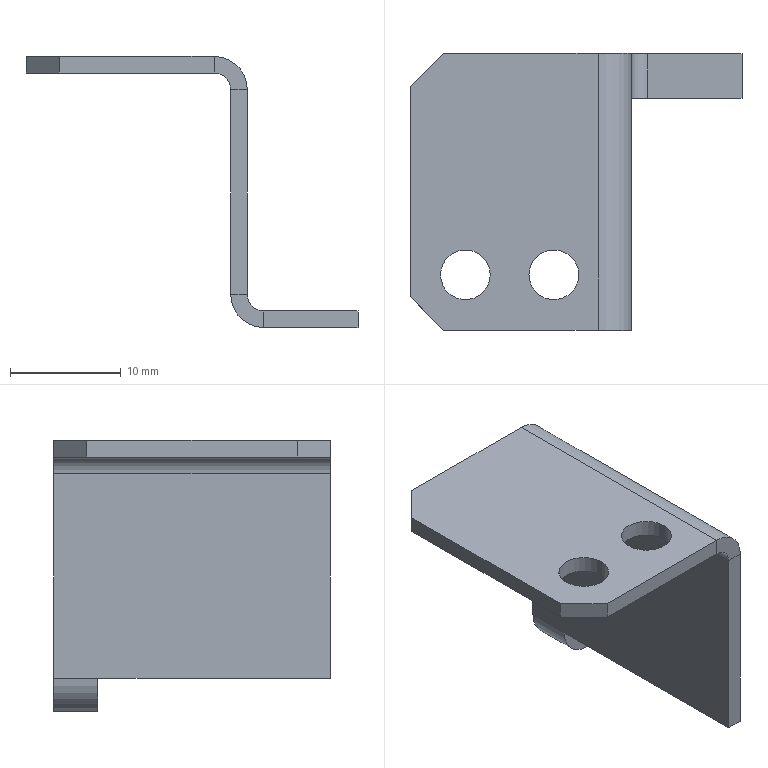Component | SolidWorks | F12529-S5109-1 | 1 solid | 29 faces | box 30 x 25 x 24.5 mm | volume 1475 mm3 | plane 21 | cylinder 8 | commonest cylinder face diameters 4.5 x4 6 x2 3 x2
STEP:
#1=CARTESIAN_POINT('',(-1.467,7.795,-1.201));
#2=VERTEX_POINT('',#1);
#3=CARTESIAN_POINT('',(-1.644,7.795,-1.201));
#4=VERTEX_POINT('',#3);
#5=CARTESIAN_POINT('',(-1.555,7.795,-1.201));
#6=DIRECTION('',(-0.,-0.,1.));
#7=DIRECTION('',(-1.,0.,-0.));
#8=AXIS2_PLACEMENT_3D('',#5,#6,#7);
#9=CIRCLE('',#8,0.08858);
#10=EDGE_CURVE('',#2,#4,#9,.T.);
#11=ORIENTED_EDGE('',*,*,#10,.T.);
#12=CARTESIAN_POINT('',(-1.644,7.795,-1.26));
#13=VERTEX_POINT('',#12);
#14=CARTESIAN_POINT('',(-1.644,7.795,-0.8661));
#15=DIRECTION('',(0.,0.,-1.));
#16=VECTOR('',#15,39.37);
#17=LINE('',#14,#16);
#18=EDGE_CURVE('',#4,#13,#17,.T.);
#19=ORIENTED_EDGE('',*,*,#18,.T.);
#20=CARTESIAN_POINT('',(-1.467,7.795,-1.26));
#21=VERTEX_POINT('',#20);
#22=CARTESIAN_POINT('',(-1.555,7.795,-1.26));
#23=DIRECTION('',(0.,0.,-1.));
#24=DIRECTION('',(1.,0.,0.));
#25=AXIS2_PLACEMENT_3D('',#22,#23,#24);
#26=CIRCLE('',#25,0.08858);
#27=EDGE_CURVE('',#13,#21,#26,.T.);
#28=ORIENTED_EDGE('',*,*,#27,.T.);
#29=CARTESIAN_POINT('',(-1.467,7.795,-0.8661));
#30=DIRECTION('',(0.,0.,-1.));
#31=VECTOR('',#30,39.37);
#32=LINE('',#29,#31);
#33=EDGE_CURVE('',#2,#21,#32,.T.);
#34=ORIENTED_EDGE('',*,*,#33,.F.);
#35=EDGE_LOOP('',(#11,#19,#28,#34));
#36=FACE_OUTER_BOUND('',#35,.T.);
#37=CARTESIAN_POINT('',(-1.555,7.795,-0.8661));
#38=DIRECTION('',(0.,0.,-1.));
#39=DIRECTION('',(1.,0.,0.));
#40=AXIS2_PLACEMENT_3D('',#37,#38,#39);
#41=CYLINDRICAL_SURFACE('',#40,0.08858);
#42=ADVANCED_FACE('',(#36),#41,.F.);
#43=CARTESIAN_POINT('',(-1.781,7.795,-1.201));
#44=VERTEX_POINT('',#43);
#45=CARTESIAN_POINT('',(-1.959,7.795,-1.201));
#46=VERTEX_POINT('',#45);
#47=CARTESIAN_POINT('',(-1.87,7.795,-1.201));
#48=DIRECTION('',(-0.,-0.,1.));
#49=DIRECTION('',(-1.,0.,-0.));
#50=AXIS2_PLACEMENT_3D('',#47,#48,#49);
#51=CIRCLE('',#50,0.08858);
#52=EDGE_CURVE('',#44,#46,#51,.T.);
#53=ORIENTED_EDGE('',*,*,#52,.T.);
#54=CARTESIAN_POINT('',(-1.959,7.795,-1.26));
#55=VERTEX_POINT('',#54);
#56=CARTESIAN_POINT('',(-1.959,7.795,-0.8661));
#57=DIRECTION('',(0.,0.,-1.));
#58=VECTOR('',#57,39.37);
#59=LINE('',#56,#58);
#60=EDGE_CURVE('',#46,#55,#59,.T.);
#61=ORIENTED_EDGE('',*,*,#60,.T.);
#62=CARTESIAN_POINT('',(-1.781,7.795,-1.26));
#63=VERTEX_POINT('',#62);
#64=CARTESIAN_POINT('',(-1.87,7.795,-1.26));
#65=DIRECTION('',(0.,0.,-1.));
#66=DIRECTION('',(1.,0.,0.));
#67=AXIS2_PLACEMENT_3D('',#64,#65,#66);
#68=CIRCLE('',#67,0.08858);
#69=EDGE_CURVE('',#55,#63,#68,.T.);
#70=ORIENTED_EDGE('',*,*,#69,.T.);
#71=CARTESIAN_POINT('',(-1.781,7.795,-0.8661));
#72=DIRECTION('',(0.,0.,-1.));
#73=VECTOR('',#72,39.37);
#74=LINE('',#71,#73);
#75=EDGE_CURVE('',#44,#63,#74,.T.);
#76=ORIENTED_EDGE('',*,*,#75,.F.);
#77=EDGE_LOOP('',(#53,#61,#70,#76));
#78=FACE_OUTER_BOUND('',#77,.T.);
#79=CARTESIAN_POINT('',(-1.87,7.795,-0.8661));
#80=DIRECTION('',(0.,0.,-1.));
#81=DIRECTION('',(1.,0.,0.));
#82=AXIS2_PLACEMENT_3D('',#79,#80,#81);
#83=CYLINDRICAL_SURFACE('',#82,0.08858);
#84=ADVANCED_FACE('',(#78),#83,.F.);
#85=CARTESIAN_POINT('',(-1.28,7.598,-1.319));
#86=VERTEX_POINT('',#85);
#87=CARTESIAN_POINT('',(-1.339,7.598,-1.319));
#88=VERTEX_POINT('',#87);
#89=CARTESIAN_POINT('',(-1.28,7.598,-1.319));
#90=DIRECTION('',(-1.,-0.,-0.));
#91=VECTOR('',#90,39.37);
#92=LINE('',#89,#91);
#93=EDGE_CURVE('',#86,#88,#92,.T.);
#94=ORIENTED_EDGE('',*,*,#93,.F.);
#95=CARTESIAN_POINT('',(-1.398,7.598,-1.201));
#96=VERTEX_POINT('',#95);
#97=CARTESIAN_POINT('',(-1.398,7.598,-1.319));
#98=DIRECTION('',(-0.,1.,-0.));
#99=DIRECTION('',(-1.,0.,0.));
#100=AXIS2_PLACEMENT_3D('',#97,#98,#99);
#101=CIRCLE('',#100,0.1181);
#102=EDGE_CURVE('',#96,#86,#101,.T.);
#103=ORIENTED_EDGE('',*,*,#102,.F.);
#104=CARTESIAN_POINT('',(-1.398,7.598,-1.26));
#105=VERTEX_POINT('',#104);
#106=CARTESIAN_POINT('',(-1.398,7.598,-1.26));
#107=DIRECTION('',(-0.,-0.,1.));
#108=VECTOR('',#107,39.37);
#109=LINE('',#106,#108);
#110=EDGE_CURVE('',#105,#96,#109,.T.);
#111=ORIENTED_EDGE('',*,*,#110,.F.);
#112=CARTESIAN_POINT('',(-1.398,7.598,-1.319));
#113=DIRECTION('',(-0.,1.,-0.));
#114=DIRECTION('',(0.,0.,-1.));
#115=AXIS2_PLACEMENT_3D('',#112,#113,#114);
#116=CIRCLE('',#115,0.05906);
#117=EDGE_CURVE('',#105,#88,#116,.T.);
#118=ORIENTED_EDGE('',*,*,#117,.T.);
#119=EDGE_LOOP('',(#94,#103,#111,#118));
#120=FACE_OUTER_BOUND('',#119,.T.);
#121=CARTESIAN_POINT('',(-1.28,7.598,-1.319));
#122=DIRECTION('',(0.,-1.,0.));
#123=DIRECTION('',(-1.,-0.,-0.));
#124=AXIS2_PLACEMENT_3D('',#121,#122,#123);
#125=PLANE('',#124);
#126=ADVANCED_FACE('',(#120),#125,.T.);
#127=CARTESIAN_POINT('',(-1.28,7.598,-2.047));
#128=VERTEX_POINT('',#127);
#129=CARTESIAN_POINT('',(-1.28,7.598,-1.201));
#130=DIRECTION('',(0.,0.,-1.));
#131=VECTOR('',#130,39.37);
#132=LINE('',#129,#131);
#133=EDGE_CURVE('',#86,#128,#132,.T.);
#134=ORIENTED_EDGE('',*,*,#133,.F.);
#135=ORIENTED_EDGE('',*,*,#93,.T.);
#136=CARTESIAN_POINT('',(-1.339,7.598,-2.047));
#137=VERTEX_POINT('',#136);
#138=CARTESIAN_POINT('',(-1.339,7.598,-1.201));
#139=DIRECTION('',(0.,0.,-1.));
#140=VECTOR('',#139,39.37);
#141=LINE('',#138,#140);
#142=EDGE_CURVE('',#88,#137,#141,.T.);
#143=ORIENTED_EDGE('',*,*,#142,.T.);
#144=CARTESIAN_POINT('',(-1.339,7.598,-2.047));
#145=DIRECTION('',(1.,0.,0.));
#146=VECTOR('',#145,39.37);
#147=LINE('',#144,#146);
#148=EDGE_CURVE('',#137,#128,#147,.T.);
#149=ORIENTED_EDGE('',*,*,#148,.T.);
#150=EDGE_LOOP('',(#134,#135,#143,#149));
#151=FACE_OUTER_BOUND('',#150,.T.);
#152=CARTESIAN_POINT('',(-1.398,7.598,-1.26));
#153=DIRECTION('',(0.,-1.,0.));
#154=DIRECTION('',(-1.,-0.,-0.));
#155=AXIS2_PLACEMENT_3D('',#152,#153,#154);
#156=PLANE('',#155);
#157=ADVANCED_FACE('',(#151),#156,.T.);
#158=CARTESIAN_POINT('',(-1.398,8.583,-1.201));
#159=VERTEX_POINT('',#158);
#160=CARTESIAN_POINT('',(-1.398,8.583,-1.26));
#161=VERTEX_POINT('',#160);
#162=CARTESIAN_POINT('',(-1.398,8.583,-1.201));
#163=DIRECTION('',(0.,0.,-1.));
#164=VECTOR('',#163,39.37);
#165=LINE('',#162,#164);
#166=EDGE_CURVE('',#159,#161,#165,.T.);
#167=ORIENTED_EDGE('',*,*,#166,.F.);
#168=CARTESIAN_POINT('',(-1.28,8.583,-1.319));
#169=VERTEX_POINT('',#168);
#170=CARTESIAN_POINT('',(-1.398,8.583,-1.319));
#171=DIRECTION('',(-0.,1.,-0.));
#172=DIRECTION('',(-1.,0.,-0.));
#173=AXIS2_PLACEMENT_3D('',#170,#171,#172);
#174=CIRCLE('',#173,0.1181);
#175=EDGE_CURVE('',#159,#169,#174,.T.);
#176=ORIENTED_EDGE('',*,*,#175,.T.);
#177=CARTESIAN_POINT('',(-1.339,8.583,-1.319));
#178=VERTEX_POINT('',#177);
#179=CARTESIAN_POINT('',(-1.339,8.583,-1.319));
#180=DIRECTION('',(1.,0.,0.));
#181=VECTOR('',#180,39.37);
#182=LINE('',#179,#181);
#183=EDGE_CURVE('',#178,#169,#182,.T.);
#184=ORIENTED_EDGE('',*,*,#183,.F.);
#185=CARTESIAN_POINT('',(-1.398,8.583,-1.319));
#186=DIRECTION('',(-0.,1.,-0.));
#187=DIRECTION('',(0.,0.,-1.));
#188=AXIS2_PLACEMENT_3D('',#185,#186,#187);
#189=CIRCLE('',#188,0.05906);
#190=EDGE_CURVE('',#161,#178,#189,.T.);
#191=ORIENTED_EDGE('',*,*,#190,.F.);
#192=EDGE_LOOP('',(#167,#176,#184,#191));
#193=FACE_OUTER_BOUND('',#192,.T.);
#194=CARTESIAN_POINT('',(-1.398,8.583,-1.201));
#195=DIRECTION('',(-0.,1.,-0.));
#196=DIRECTION('',(1.,0.,0.));
#197=AXIS2_PLACEMENT_3D('',#194,#195,#196);
#198=PLANE('',#197);
#199=ADVANCED_FACE('',(#193),#198,.T.);
#200=CARTESIAN_POINT('',(-1.949,8.583,-1.26));
#201=VERTEX_POINT('',#200);
#202=CARTESIAN_POINT('',(-2.067,8.583,-1.26));
#203=DIRECTION('',(1.,0.,0.));
#204=VECTOR('',#203,39.37);
#205=LINE('',#202,#204);
#206=EDGE_CURVE('',#201,#161,#205,.T.);
#207=ORIENTED_EDGE('',*,*,#206,.F.);
#208=CARTESIAN_POINT('',(-1.949,8.583,-1.201));
#209=VERTEX_POINT('',#208);
#210=CARTESIAN_POINT('',(-1.949,8.583,-1.319));
#211=DIRECTION('',(-0.,-0.,1.));
#212=VECTOR('',#211,39.37);
#213=LINE('',#210,#212);
#214=EDGE_CURVE('',#201,#209,#213,.T.);
#215=ORIENTED_EDGE('',*,*,#214,.T.);
#216=CARTESIAN_POINT('',(-2.067,8.583,-1.201));
#217=DIRECTION('',(1.,0.,0.));
#218=VECTOR('',#217,39.37);
#219=LINE('',#216,#218);
#220=EDGE_CURVE('',#209,#159,#219,.T.);
#221=ORIENTED_EDGE('',*,*,#220,.T.);
#222=ORIENTED_EDGE('',*,*,#166,.T.);
#223=EDGE_LOOP('',(#207,#215,#221,#222));
#224=FACE_OUTER_BOUND('',#223,.T.);
#225=CARTESIAN_POINT('',(-1.339,8.583,-1.319));
#226=DIRECTION('',(-0.,1.,-0.));
#227=DIRECTION('',(1.,0.,0.));
#228=AXIS2_PLACEMENT_3D('',#225,#226,#227);
#229=PLANE('',#228);
#230=ADVANCED_FACE('',(#224),#229,.T.);
#231=CARTESIAN_POINT('',(-1.28,8.583,-2.047));
#232=VERTEX_POINT('',#231);
#233=CARTESIAN_POINT('',(-1.28,8.583,-1.201));
#234=DIRECTION('',(0.,0.,-1.));
#235=VECTOR('',#234,39.37);
#236=LINE('',#233,#235);
#237=EDGE_CURVE('',#169,#232,#236,.T.);
#238=ORIENTED_EDGE('',*,*,#237,.T.);
#239=CARTESIAN_POINT('',(-1.339,8.583,-2.047));
#240=VERTEX_POINT('',#239);
#241=CARTESIAN_POINT('',(-1.28,8.583,-2.047));
#242=DIRECTION('',(-1.,-0.,-0.));
#243=VECTOR('',#242,39.37);
#244=LINE('',#241,#243);
#245=EDGE_CURVE('',#232,#240,#244,.T.);
#246=ORIENTED_EDGE('',*,*,#245,.T.);
#247=CARTESIAN_POINT('',(-1.339,8.583,-1.201));
#248=DIRECTION('',(0.,0.,-1.));
#249=VECTOR('',#248,39.37);
#250=LINE('',#247,#249);
#251=EDGE_CURVE('',#178,#240,#250,.T.);
#252=ORIENTED_EDGE('',*,*,#251,.F.);
#253=ORIENTED_EDGE('',*,*,#183,.T.);
#254=EDGE_LOOP('',(#238,#246,#252,#253));
#255=FACE_OUTER_BOUND('',#254,.T.);
#256=CARTESIAN_POINT('',(-1.22,8.583,-2.165));
#257=DIRECTION('',(-0.,1.,-0.));
#258=DIRECTION('',(1.,0.,0.));
#259=AXIS2_PLACEMENT_3D('',#256,#257,#258);
#260=PLANE('',#259);
#261=ADVANCED_FACE('',(#255),#260,.T.);
#262=ORIENTED_EDGE('',*,*,#237,.F.);
#263=CARTESIAN_POINT('',(-1.28,7.598,-1.319));
#264=DIRECTION('',(-0.,1.,-0.));
#265=VECTOR('',#264,39.37);
#266=LINE('',#263,#265);
#267=EDGE_CURVE('',#86,#169,#266,.T.);
#268=ORIENTED_EDGE('',*,*,#267,.F.);
#269=ORIENTED_EDGE('',*,*,#133,.T.);
#270=CARTESIAN_POINT('',(-1.28,8.425,-2.047));
#271=VERTEX_POINT('',#270);
#272=CARTESIAN_POINT('',(-1.28,7.598,-2.047));
#273=DIRECTION('',(-0.,1.,-0.));
#274=VECTOR('',#273,39.37);
#275=LINE('',#272,#274);
#276=EDGE_CURVE('',#128,#271,#275,.T.);
#277=ORIENTED_EDGE('',*,*,#276,.T.);
#278=CARTESIAN_POINT('',(-1.28,7.598,-2.047));
#279=DIRECTION('',(-0.,1.,-0.));
#280=VECTOR('',#279,39.37);
#281=LINE('',#278,#280);
#282=EDGE_CURVE('',#271,#232,#281,.T.);
#283=ORIENTED_EDGE('',*,*,#282,.T.);
#284=EDGE_LOOP('',(#262,#268,#269,#277,#283));
#285=FACE_OUTER_BOUND('',#284,.T.);
#286=CARTESIAN_POINT('',(-1.28,7.598,-1.201));
#287=DIRECTION('',(1.,0.,0.));
#288=DIRECTION('',(-0.,-0.,1.));
#289=AXIS2_PLACEMENT_3D('',#286,#287,#288);
#290=PLANE('',#289);
#291=ADVANCED_FACE('',(#285),#290,.T.);
#292=ORIENTED_EDGE('',*,*,#175,.F.);
#293=CARTESIAN_POINT('',(-1.398,7.598,-1.201));
#294=DIRECTION('',(-0.,1.,-0.));
#295=VECTOR('',#294,39.37);
#296=LINE('',#293,#295);
#297=EDGE_CURVE('',#96,#159,#296,.T.);
#298=ORIENTED_EDGE('',*,*,#297,.F.);
#299=ORIENTED_EDGE('',*,*,#102,.T.);
#300=ORIENTED_EDGE('',*,*,#267,.T.);
#301=EDGE_LOOP('',(#292,#298,#299,#300));
#302=FACE_OUTER_BOUND('',#301,.T.);
#303=CARTESIAN_POINT('',(-1.398,7.598,-1.319));
#304=DIRECTION('',(-0.,1.,-0.));
#305=DIRECTION('',(1.,0.,0.));
#306=AXIS2_PLACEMENT_3D('',#303,#304,#305);
#307=CYLINDRICAL_SURFACE('',#306,0.1181);
#308=ADVANCED_FACE('',(#302),#307,.T.);
#309=ORIENTED_EDGE('',*,*,#10,.F.);
#310=CARTESIAN_POINT('',(-1.555,7.795,-1.201));
#311=DIRECTION('',(-0.,-0.,1.));
#312=DIRECTION('',(-1.,0.,-0.));
#313=AXIS2_PLACEMENT_3D('',#310,#311,#312);
#314=CIRCLE('',#313,0.08858);
#315=EDGE_CURVE('',#4,#2,#314,.T.);
#316=ORIENTED_EDGE('',*,*,#315,.F.);
#317=EDGE_LOOP('',(#309,#316));
#318=FACE_BOUND('',#317,.T.);
#319=ORIENTED_EDGE('',*,*,#52,.F.);
#320=CARTESIAN_POINT('',(-1.87,7.795,-1.201));
#321=DIRECTION('',(-0.,-0.,1.));
#322=DIRECTION('',(-1.,0.,-0.));
#323=AXIS2_PLACEMENT_3D('',#320,#321,#322);
#324=CIRCLE('',#323,0.08858);
#325=EDGE_CURVE('',#46,#44,#324,.T.);
#326=ORIENTED_EDGE('',*,*,#325,.F.);
#327=EDGE_LOOP('',(#319,#326));
#328=FACE_BOUND('',#327,.T.);
#329=ORIENTED_EDGE('',*,*,#220,.F.);
#330=CARTESIAN_POINT('',(-2.067,8.465,-1.201));
#331=VERTEX_POINT('',#330);
#332=CARTESIAN_POINT('',(-2.5,8.031,-1.201));
#333=DIRECTION('',(-0.7071,-0.7071,-0.));
#334=VECTOR('',#333,39.37);
#335=LINE('',#332,#334);
#336=EDGE_CURVE('',#209,#331,#335,.T.);
#337=ORIENTED_EDGE('',*,*,#336,.T.);
#338=CARTESIAN_POINT('',(-2.067,7.717,-1.201));
#339=VERTEX_POINT('',#338);
#340=CARTESIAN_POINT('',(-2.067,7.598,-1.201));
#341=DIRECTION('',(-0.,1.,-0.));
#342=VECTOR('',#341,39.37);
#343=LINE('',#340,#342);
#344=EDGE_CURVE('',#339,#331,#343,.T.);
#345=ORIENTED_EDGE('',*,*,#344,.F.);
#346=CARTESIAN_POINT('',(-1.949,7.598,-1.201));
#347=VERTEX_POINT('',#346);
#348=CARTESIAN_POINT('',(-2.008,7.657,-1.201));
#349=DIRECTION('',(0.7071,-0.7071,0.));
#350=VECTOR('',#349,39.37);
#351=LINE('',#348,#350);
#352=EDGE_CURVE('',#339,#347,#351,.T.);
#353=ORIENTED_EDGE('',*,*,#352,.T.);
#354=CARTESIAN_POINT('',(-2.067,7.598,-1.201));
#355=DIRECTION('',(1.,0.,0.));
#356=VECTOR('',#355,39.37);
#357=LINE('',#354,#356);
#358=EDGE_CURVE('',#347,#96,#357,.T.);
#359=ORIENTED_EDGE('',*,*,#358,.T.);
#360=ORIENTED_EDGE('',*,*,#297,.T.);
#361=EDGE_LOOP('',(#329,#337,#345,#353,#359,#360));
#362=FACE_OUTER_BOUND('',#361,.T.);
#363=CARTESIAN_POINT('',(-2.067,7.598,-1.201));
#364=DIRECTION('',(-0.,-0.,1.));
#365=DIRECTION('',(-1.,-0.,-0.));
#366=AXIS2_PLACEMENT_3D('',#363,#364,#365);
#367=PLANE('',#366);
#368=ADVANCED_FACE('',(#318,#328,#362),#367,.T.);
#369=ORIENTED_EDGE('',*,*,#344,.T.);
#370=CARTESIAN_POINT('',(-2.067,8.465,-1.26));
#371=VERTEX_POINT('',#370);
#372=CARTESIAN_POINT('',(-2.067,8.465,-1.26));
#373=DIRECTION('',(0.,0.,-1.));
#374=VECTOR('',#373,39.37);
#375=LINE('',#372,#374);
#376=EDGE_CURVE('',#331,#371,#375,.T.);
#377=ORIENTED_EDGE('',*,*,#376,.T.);
#378=CARTESIAN_POINT('',(-2.067,7.717,-1.26));
#379=VERTEX_POINT('',#378);
#380=CARTESIAN_POINT('',(-2.067,7.598,-1.26));
#381=DIRECTION('',(-0.,1.,-0.));
#382=VECTOR('',#381,39.37);
#383=LINE('',#380,#382);
#384=EDGE_CURVE('',#379,#371,#383,.T.);
#385=ORIENTED_EDGE('',*,*,#384,.F.);
#386=CARTESIAN_POINT('',(-2.067,7.717,-1.201));
#387=DIRECTION('',(-0.,-0.,1.));
#388=VECTOR('',#387,39.37);
#389=LINE('',#386,#388);
#390=EDGE_CURVE('',#379,#339,#389,.T.);
#391=ORIENTED_EDGE('',*,*,#390,.T.);
#392=EDGE_LOOP('',(#369,#377,#385,#391));
#393=FACE_OUTER_BOUND('',#392,.T.);
#394=CARTESIAN_POINT('',(-2.067,7.598,-1.26));
#395=DIRECTION('',(-1.,-0.,-0.));
#396=DIRECTION('',(0.,0.,-1.));
#397=AXIS2_PLACEMENT_3D('',#394,#395,#396);
#398=PLANE('',#397);
#399=ADVANCED_FACE('',(#393),#398,.T.);
#400=CARTESIAN_POINT('',(-1.555,7.795,-1.26));
#401=DIRECTION('',(0.,0.,-1.));
#402=DIRECTION('',(1.,0.,0.));
#403=AXIS2_PLACEMENT_3D('',#400,#401,#402);
#404=CIRCLE('',#403,0.08858);
#405=EDGE_CURVE('',#21,#13,#404,.T.);
#406=ORIENTED_EDGE('',*,*,#405,.F.);
#407=ORIENTED_EDGE('',*,*,#27,.F.);
#408=EDGE_LOOP('',(#406,#407));
#409=FACE_BOUND('',#408,.T.);
#410=CARTESIAN_POINT('',(-1.87,7.795,-1.26));
#411=DIRECTION('',(0.,0.,-1.));
#412=DIRECTION('',(1.,0.,0.));
#413=AXIS2_PLACEMENT_3D('',#410,#411,#412);
#414=CIRCLE('',#413,0.08858);
#415=EDGE_CURVE('',#63,#55,#414,.T.);
#416=ORIENTED_EDGE('',*,*,#415,.F.);
#417=ORIENTED_EDGE('',*,*,#69,.F.);
#418=EDGE_LOOP('',(#416,#417));
#419=FACE_BOUND('',#418,.T.);
#420=ORIENTED_EDGE('',*,*,#384,.T.);
#421=CARTESIAN_POINT('',(-1.949,8.583,-1.26));
#422=DIRECTION('',(0.7071,0.7071,0.));
#423=VECTOR('',#422,39.37);
#424=LINE('',#421,#423);
#425=EDGE_CURVE('',#371,#201,#424,.T.);
#426=ORIENTED_EDGE('',*,*,#425,.T.);
#427=ORIENTED_EDGE('',*,*,#206,.T.);
#428=CARTESIAN_POINT('',(-1.398,7.598,-1.26));
#429=DIRECTION('',(-0.,1.,-0.));
#430=VECTOR('',#429,39.37);
#431=LINE('',#428,#430);
#432=EDGE_CURVE('',#105,#161,#431,.T.);
#433=ORIENTED_EDGE('',*,*,#432,.F.);
#434=CARTESIAN_POINT('',(-1.949,7.598,-1.26));
#435=VERTEX_POINT('',#434);
#436=CARTESIAN_POINT('',(-2.067,7.598,-1.26));
#437=DIRECTION('',(1.,0.,0.));
#438=VECTOR('',#437,39.37);
#439=LINE('',#436,#438);
#440=EDGE_CURVE('',#435,#105,#439,.T.);
#441=ORIENTED_EDGE('',*,*,#440,.F.);
#442=CARTESIAN_POINT('',(-2.067,7.717,-1.26));
#443=DIRECTION('',(-0.7071,0.7071,-0.));
#444=VECTOR('',#443,39.37);
#445=LINE('',#442,#444);
#446=EDGE_CURVE('',#435,#379,#445,.T.);
#447=ORIENTED_EDGE('',*,*,#446,.T.);
#448=EDGE_LOOP('',(#420,#426,#427,#433,#441,#447));
#449=FACE_OUTER_BOUND('',#448,.T.);
#450=CARTESIAN_POINT('',(-2.067,7.598,-1.26));
#451=DIRECTION('',(-0.,-0.,1.));
#452=DIRECTION('',(-1.,-0.,-0.));
#453=AXIS2_PLACEMENT_3D('',#450,#451,#452);
#454=PLANE('',#453);
#455=ADVANCED_FACE('',(#409,#419,#449),#454,.F.);
#456=ORIENTED_EDGE('',*,*,#190,.T.);
#457=CARTESIAN_POINT('',(-1.339,7.598,-1.319));
#458=DIRECTION('',(-0.,1.,-0.));
#459=VECTOR('',#458,39.37);
#460=LINE('',#457,#459);
#461=EDGE_CURVE('',#88,#178,#460,.T.);
#462=ORIENTED_EDGE('',*,*,#461,.F.);
#463=ORIENTED_EDGE('',*,*,#117,.F.);
#464=ORIENTED_EDGE('',*,*,#432,.T.);
#465=EDGE_LOOP('',(#456,#462,#463,#464));
#466=FACE_OUTER_BOUND('',#465,.T.);
#467=CARTESIAN_POINT('',(-1.398,7.598,-1.319));
#468=DIRECTION('',(-0.,1.,-0.));
#469=DIRECTION('',(1.,0.,0.));
#470=AXIS2_PLACEMENT_3D('',#467,#468,#469);
#471=CYLINDRICAL_SURFACE('',#470,0.05906);
#472=ADVANCED_FACE('',(#466),#471,.F.);
#473=ORIENTED_EDGE('',*,*,#251,.T.);
#474=CARTESIAN_POINT('',(-1.339,8.425,-2.047));
#475=VERTEX_POINT('',#474);
#476=CARTESIAN_POINT('',(-1.339,7.598,-2.047));
#477=DIRECTION('',(-0.,1.,-0.));
#478=VECTOR('',#477,39.37);
#479=LINE('',#476,#478);
#480=EDGE_CURVE('',#475,#240,#479,.T.);
#481=ORIENTED_EDGE('',*,*,#480,.F.);
#482=CARTESIAN_POINT('',(-1.339,7.598,-2.047));
#483=DIRECTION('',(-0.,1.,-0.));
#484=VECTOR('',#483,39.37);
#485=LINE('',#482,#484);
#486=EDGE_CURVE('',#137,#475,#485,.T.);
#487=ORIENTED_EDGE('',*,*,#486,.F.);
#488=ORIENTED_EDGE('',*,*,#142,.F.);
#489=ORIENTED_EDGE('',*,*,#461,.T.);
#490=EDGE_LOOP('',(#473,#481,#487,#488,#489));
#491=FACE_OUTER_BOUND('',#490,.T.);
#492=CARTESIAN_POINT('',(-1.339,7.598,-1.201));
#493=DIRECTION('',(1.,0.,0.));
#494=DIRECTION('',(-0.,-0.,1.));
#495=AXIS2_PLACEMENT_3D('',#492,#493,#494);
#496=PLANE('',#495);
#497=ADVANCED_FACE('',(#491),#496,.F.);
#498=ORIENTED_EDGE('',*,*,#358,.F.);
#499=CARTESIAN_POINT('',(-1.949,7.598,-1.26));
#500=DIRECTION('',(0.,0.,-1.));
#501=VECTOR('',#500,39.37);
#502=LINE('',#499,#501);
#503=EDGE_CURVE('',#347,#435,#502,.T.);
#504=ORIENTED_EDGE('',*,*,#503,.T.);
#505=ORIENTED_EDGE('',*,*,#440,.T.);
#506=ORIENTED_EDGE('',*,*,#110,.T.);
#507=EDGE_LOOP('',(#498,#504,#505,#506));
#508=FACE_OUTER_BOUND('',#507,.T.);
#509=CARTESIAN_POINT('',(-1.22,7.598,-2.047));
#510=DIRECTION('',(-0.,1.,-0.));
#511=DIRECTION('',(-0.,-0.,1.));
#512=AXIS2_PLACEMENT_3D('',#509,#510,#511);
#513=PLANE('',#512);
#514=ADVANCED_FACE('',(#508),#513,.F.);
#515=ORIENTED_EDGE('',*,*,#425,.F.);
#516=ORIENTED_EDGE('',*,*,#376,.F.);
#517=ORIENTED_EDGE('',*,*,#336,.F.);
#518=ORIENTED_EDGE('',*,*,#214,.F.);
#519=EDGE_LOOP('',(#515,#516,#517,#518));
#520=FACE_OUTER_BOUND('',#519,.T.);
#521=CARTESIAN_POINT('',(-1.949,8.583,-1.319));
#522=DIRECTION('',(0.7071,-0.7071,0.));
#523=DIRECTION('',(-0.7071,-0.7071,-0.));
#524=AXIS2_PLACEMENT_3D('',#521,#522,#523);
#525=PLANE('',#524);
#526=ADVANCED_FACE('',(#520),#525,.F.);
#527=ORIENTED_EDGE('',*,*,#446,.F.);
#528=ORIENTED_EDGE('',*,*,#503,.F.);
#529=ORIENTED_EDGE('',*,*,#352,.F.);
#530=ORIENTED_EDGE('',*,*,#390,.F.);
#531=EDGE_LOOP('',(#527,#528,#529,#530));
#532=FACE_OUTER_BOUND('',#531,.T.);
#533=CARTESIAN_POINT('',(-2.067,7.717,-1.26));
#534=DIRECTION('',(-0.7071,-0.7071,-0.));
#535=DIRECTION('',(-0.7071,0.7071,-0.));
#536=AXIS2_PLACEMENT_3D('',#533,#534,#535);
#537=PLANE('',#536);
#538=ADVANCED_FACE('',(#532),#537,.T.);
#539=ORIENTED_EDGE('',*,*,#486,.T.);
#540=CARTESIAN_POINT('',(-1.28,8.425,-2.047));
#541=DIRECTION('',(-1.,-0.,-0.));
#542=VECTOR('',#541,39.37);
#543=LINE('',#540,#542);
#544=EDGE_CURVE('',#271,#475,#543,.T.);
#545=ORIENTED_EDGE('',*,*,#544,.F.);
#546=ORIENTED_EDGE('',*,*,#276,.F.);
#547=ORIENTED_EDGE('',*,*,#148,.F.);
#548=EDGE_LOOP('',(#539,#545,#546,#547));
#549=FACE_OUTER_BOUND('',#548,.T.);
#550=CARTESIAN_POINT('',(-1.28,7.598,-2.047));
#551=DIRECTION('',(-0.,-0.,1.));
#552=DIRECTION('',(-1.,-0.,-0.));
#553=AXIS2_PLACEMENT_3D('',#550,#551,#552);
#554=PLANE('',#553);
#555=ADVANCED_FACE('',(#549),#554,.F.);
#556=ORIENTED_EDGE('',*,*,#544,.T.);
#557=CARTESIAN_POINT('',(-1.22,8.425,-2.165));
#558=VERTEX_POINT('',#557);
#559=CARTESIAN_POINT('',(-1.22,8.425,-2.047));
#560=DIRECTION('',(0.,-1.,0.));
#561=DIRECTION('',(1.,0.,0.));
#562=AXIS2_PLACEMENT_3D('',#559,#560,#561);
#563=CIRCLE('',#562,0.1181);
#564=EDGE_CURVE('',#475,#558,#563,.T.);
#565=ORIENTED_EDGE('',*,*,#564,.T.);
#566=CARTESIAN_POINT('',(-1.22,8.425,-2.106));
#567=VERTEX_POINT('',#566);
#568=CARTESIAN_POINT('',(-1.22,8.425,-2.165));
#569=DIRECTION('',(-0.,-0.,1.));
#570=VECTOR('',#569,39.37);
#571=LINE('',#568,#570);
#572=EDGE_CURVE('',#558,#567,#571,.T.);
#573=ORIENTED_EDGE('',*,*,#572,.T.);
#574=CARTESIAN_POINT('',(-1.22,8.425,-2.047));
#575=DIRECTION('',(0.,-1.,0.));
#576=DIRECTION('',(-1.,0.,0.));
#577=AXIS2_PLACEMENT_3D('',#574,#575,#576);
#578=CIRCLE('',#577,0.05906);
#579=EDGE_CURVE('',#271,#567,#578,.T.);
#580=ORIENTED_EDGE('',*,*,#579,.F.);
#581=EDGE_LOOP('',(#556,#565,#573,#580));
#582=FACE_OUTER_BOUND('',#581,.T.);
#583=CARTESIAN_POINT('',(-1.22,8.425,-2.047));
#584=DIRECTION('',(-0.,1.,-0.));
#585=DIRECTION('',(1.,0.,0.));
#586=AXIS2_PLACEMENT_3D('',#583,#584,#585);
#587=PLANE('',#586);
#588=ADVANCED_FACE('',(#582),#587,.F.);
#589=CARTESIAN_POINT('',(-1.22,8.583,-2.165));
#590=VERTEX_POINT('',#589);
#591=CARTESIAN_POINT('',(-1.22,8.583,-2.106));
#592=VERTEX_POINT('',#591);
#593=CARTESIAN_POINT('',(-1.22,8.583,-2.165));
#594=DIRECTION('',(-0.,-0.,1.));
#595=VECTOR('',#594,39.37);
#596=LINE('',#593,#595);
#597=EDGE_CURVE('',#590,#592,#596,.T.);
#598=ORIENTED_EDGE('',*,*,#597,.F.);
#599=CARTESIAN_POINT('',(-1.22,8.583,-2.047));
#600=DIRECTION('',(-0.,1.,-0.));
#601=DIRECTION('',(1.,0.,0.));
#602=AXIS2_PLACEMENT_3D('',#599,#600,#601);
#603=CIRCLE('',#602,0.1181);
#604=EDGE_CURVE('',#590,#240,#603,.T.);
#605=ORIENTED_EDGE('',*,*,#604,.T.);
#606=ORIENTED_EDGE('',*,*,#245,.F.);
#607=CARTESIAN_POINT('',(-1.22,8.583,-2.047));
#608=DIRECTION('',(-0.,1.,-0.));
#609=DIRECTION('',(1.,0.,0.));
#610=AXIS2_PLACEMENT_3D('',#607,#608,#609);
#611=CIRCLE('',#610,0.05906);
#612=EDGE_CURVE('',#592,#232,#611,.T.);
#613=ORIENTED_EDGE('',*,*,#612,.F.);
#614=EDGE_LOOP('',(#598,#605,#606,#613));
#615=FACE_OUTER_BOUND('',#614,.T.);
#616=CARTESIAN_POINT('',(-1.22,8.583,-2.047));
#617=DIRECTION('',(0.,-1.,0.));
#618=DIRECTION('',(-1.,-0.,-0.));
#619=AXIS2_PLACEMENT_3D('',#616,#617,#618);
#620=PLANE('',#619);
#621=ADVANCED_FACE('',(#615),#620,.F.);
#622=ORIENTED_EDGE('',*,*,#612,.T.);
#623=ORIENTED_EDGE('',*,*,#282,.F.);
#624=ORIENTED_EDGE('',*,*,#579,.T.);
#625=CARTESIAN_POINT('',(-1.22,7.598,-2.106));
#626=DIRECTION('',(-0.,1.,-0.));
#627=VECTOR('',#626,39.37);
#628=LINE('',#625,#627);
#629=EDGE_CURVE('',#567,#592,#628,.T.);
#630=ORIENTED_EDGE('',*,*,#629,.T.);
#631=EDGE_LOOP('',(#622,#623,#624,#630));
#632=FACE_OUTER_BOUND('',#631,.T.);
#633=CARTESIAN_POINT('',(-1.22,8.286,-2.047));
#634=DIRECTION('',(-0.,1.,-0.));
#635=DIRECTION('',(1.,0.,0.));
#636=AXIS2_PLACEMENT_3D('',#633,#634,#635);
#637=CYLINDRICAL_SURFACE('',#636,0.05906);
#638=ADVANCED_FACE('',(#632),#637,.F.);
#639=ORIENTED_EDGE('',*,*,#604,.F.);
#640=CARTESIAN_POINT('',(-1.22,7.598,-2.165));
#641=DIRECTION('',(-0.,1.,-0.));
#642=VECTOR('',#641,39.37);
#643=LINE('',#640,#642);
#644=EDGE_CURVE('',#558,#590,#643,.T.);
#645=ORIENTED_EDGE('',*,*,#644,.F.);
#646=ORIENTED_EDGE('',*,*,#564,.F.);
#647=ORIENTED_EDGE('',*,*,#480,.T.);
#648=EDGE_LOOP('',(#639,#645,#646,#647));
#649=FACE_OUTER_BOUND('',#648,.T.);
#650=CARTESIAN_POINT('',(-1.22,8.286,-2.047));
#651=DIRECTION('',(-0.,1.,-0.));
#652=DIRECTION('',(1.,0.,0.));
#653=AXIS2_PLACEMENT_3D('',#650,#651,#652);
#654=CYLINDRICAL_SURFACE('',#653,0.1181);
#655=ADVANCED_FACE('',(#649),#654,.T.);
#656=CARTESIAN_POINT('',(-0.8858,8.425,-2.106));
#657=VERTEX_POINT('',#656);
#658=CARTESIAN_POINT('',(-0.8858,8.425,-2.165));
#659=VERTEX_POINT('',#658);
#660=CARTESIAN_POINT('',(-0.8858,8.425,-2.106));
#661=DIRECTION('',(0.,0.,-1.));
#662=VECTOR('',#661,39.37);
#663=LINE('',#660,#662);
#664=EDGE_CURVE('',#657,#659,#663,.T.);
#665=ORIENTED_EDGE('',*,*,#664,.T.);
#666=CARTESIAN_POINT('',(-0.8858,8.583,-2.165));
#667=VERTEX_POINT('',#666);
#668=CARTESIAN_POINT('',(-0.8858,7.598,-2.165));
#669=DIRECTION('',(-0.,1.,-0.));
#670=VECTOR('',#669,39.37);
#671=LINE('',#668,#670);
#672=EDGE_CURVE('',#659,#667,#671,.T.);
#673=ORIENTED_EDGE('',*,*,#672,.T.);
#674=CARTESIAN_POINT('',(-0.8858,8.583,-2.106));
#675=VERTEX_POINT('',#674);
#676=CARTESIAN_POINT('',(-0.8858,8.583,-2.106));
#677=DIRECTION('',(0.,0.,-1.));
#678=VECTOR('',#677,39.37);
#679=LINE('',#676,#678);
#680=EDGE_CURVE('',#675,#667,#679,.T.);
#681=ORIENTED_EDGE('',*,*,#680,.F.);
#682=CARTESIAN_POINT('',(-0.8858,7.598,-2.106));
#683=DIRECTION('',(-0.,1.,-0.));
#684=VECTOR('',#683,39.37);
#685=LINE('',#682,#684);
#686=EDGE_CURVE('',#657,#675,#685,.T.);
#687=ORIENTED_EDGE('',*,*,#686,.F.);
#688=EDGE_LOOP('',(#665,#673,#681,#687));
#689=FACE_OUTER_BOUND('',#688,.T.);
#690=CARTESIAN_POINT('',(-0.8858,7.598,-2.106));
#691=DIRECTION('',(1.,0.,0.));
#692=DIRECTION('',(-0.,-0.,1.));
#693=AXIS2_PLACEMENT_3D('',#690,#691,#692);
#694=PLANE('',#693);
#695=ADVANCED_FACE('',(#689),#694,.T.);
#696=CARTESIAN_POINT('',(-0.8858,8.425,-2.106));
#697=DIRECTION('',(1.,0.,0.));
#698=VECTOR('',#697,39.37);
#699=LINE('',#696,#698);
#700=EDGE_CURVE('',#567,#657,#699,.T.);
#701=ORIENTED_EDGE('',*,*,#700,.T.);
#702=ORIENTED_EDGE('',*,*,#686,.T.);
#703=CARTESIAN_POINT('',(-1.28,8.583,-2.106));
#704=DIRECTION('',(1.,0.,0.));
#705=VECTOR('',#704,39.37);
#706=LINE('',#703,#705);
#707=EDGE_CURVE('',#592,#675,#706,.T.);
#708=ORIENTED_EDGE('',*,*,#707,.F.);
#709=ORIENTED_EDGE('',*,*,#629,.F.);
#710=EDGE_LOOP('',(#701,#702,#708,#709));
#711=FACE_OUTER_BOUND('',#710,.T.);
#712=CARTESIAN_POINT('',(-1.28,7.598,-2.106));
#713=DIRECTION('',(-0.,-0.,1.));
#714=DIRECTION('',(-1.,-0.,-0.));
#715=AXIS2_PLACEMENT_3D('',#712,#713,#714);
#716=PLANE('',#715);
#717=ADVANCED_FACE('',(#711),#716,.T.);
#718=ORIENTED_EDGE('',*,*,#572,.F.);
#719=CARTESIAN_POINT('',(-1.28,8.425,-2.165));
#720=DIRECTION('',(-1.,-0.,-0.));
#721=VECTOR('',#720,39.37);
#722=LINE('',#719,#721);
#723=EDGE_CURVE('',#659,#558,#722,.T.);
#724=ORIENTED_EDGE('',*,*,#723,.F.);
#725=ORIENTED_EDGE('',*,*,#664,.F.);
#726=ORIENTED_EDGE('',*,*,#700,.F.);
#727=EDGE_LOOP('',(#718,#724,#725,#726));
#728=FACE_OUTER_BOUND('',#727,.T.);
#729=CARTESIAN_POINT('',(-0.8858,8.425,-2.106));
#730=DIRECTION('',(-0.,1.,-0.));
#731=DIRECTION('',(-0.,-0.,1.));
#732=AXIS2_PLACEMENT_3D('',#729,#730,#731);
#733=PLANE('',#732);
#734=ADVANCED_FACE('',(#728),#733,.F.);
#735=ORIENTED_EDGE('',*,*,#672,.F.);
#736=ORIENTED_EDGE('',*,*,#723,.T.);
#737=ORIENTED_EDGE('',*,*,#644,.T.);
#738=CARTESIAN_POINT('',(-1.28,8.583,-2.165));
#739=DIRECTION('',(1.,0.,0.));
#740=VECTOR('',#739,39.37);
#741=LINE('',#738,#740);
#742=EDGE_CURVE('',#590,#667,#741,.T.);
#743=ORIENTED_EDGE('',*,*,#742,.T.);
#744=EDGE_LOOP('',(#735,#736,#737,#743));
#745=FACE_OUTER_BOUND('',#744,.T.);
#746=CARTESIAN_POINT('',(-1.28,7.598,-2.165));
#747=DIRECTION('',(-0.,-0.,1.));
#748=DIRECTION('',(-1.,-0.,-0.));
#749=AXIS2_PLACEMENT_3D('',#746,#747,#748);
#750=PLANE('',#749);
#751=ADVANCED_FACE('',(#745),#750,.F.);
#752=ORIENTED_EDGE('',*,*,#742,.F.);
#753=ORIENTED_EDGE('',*,*,#597,.T.);
#754=ORIENTED_EDGE('',*,*,#707,.T.);
#755=ORIENTED_EDGE('',*,*,#680,.T.);
#756=EDGE_LOOP('',(#752,#753,#754,#755));
#757=FACE_OUTER_BOUND('',#756,.T.);
#758=CARTESIAN_POINT('',(-1.22,8.583,-2.047));
#759=DIRECTION('',(-0.,1.,-0.));
#760=DIRECTION('',(-0.,-0.,1.));
#761=AXIS2_PLACEMENT_3D('',#758,#759,#760);
#762=PLANE('',#761);
#763=ADVANCED_FACE('',(#757),#762,.T.);
#764=ORIENTED_EDGE('',*,*,#60,.F.);
#765=ORIENTED_EDGE('',*,*,#325,.T.);
#766=ORIENTED_EDGE('',*,*,#75,.T.);
#767=ORIENTED_EDGE('',*,*,#415,.T.);
#768=EDGE_LOOP('',(#764,#765,#766,#767));
#769=FACE_OUTER_BOUND('',#768,.T.);
#770=CARTESIAN_POINT('',(-1.87,7.795,-0.8661));
#771=DIRECTION('',(0.,0.,-1.));
#772=DIRECTION('',(1.,0.,0.));
#773=AXIS2_PLACEMENT_3D('',#770,#771,#772);
#774=CYLINDRICAL_SURFACE('',#773,0.08858);
#775=ADVANCED_FACE('',(#769),#774,.F.);
#776=ORIENTED_EDGE('',*,*,#18,.F.);
#777=ORIENTED_EDGE('',*,*,#315,.T.);
#778=ORIENTED_EDGE('',*,*,#33,.T.);
#779=ORIENTED_EDGE('',*,*,#405,.T.);
#780=EDGE_LOOP('',(#776,#777,#778,#779));
#781=FACE_OUTER_BOUND('',#780,.T.);
#782=CARTESIAN_POINT('',(-1.555,7.795,-0.8661));
#783=DIRECTION('',(0.,0.,-1.));
#784=DIRECTION('',(1.,0.,0.));
#785=AXIS2_PLACEMENT_3D('',#782,#783,#784);
#786=CYLINDRICAL_SURFACE('',#785,0.08858);
#787=ADVANCED_FACE('',(#781),#786,.F.);
#788=CLOSED_SHELL('',(#42,#84,#126,#157,#199,#230,#261,#291,#308,#368,#399,#455,#472,#497,#514,#526,#538,#555,#588,#621,#638,#655,#695,#717,#734,#751,#763,#775,#787));
#789=MANIFOLD_SOLID_BREP('',#788);
#790=CARTESIAN_POINT('',(0.,0.,0.));
#791=DIRECTION('',(0.,0.,1.));
#792=DIRECTION('',(1.,0.,0.));
#793=AXIS2_PLACEMENT_3D('',#790,#791,#792);
#794=(LENGTH_UNIT()NAMED_UNIT(*)SI_UNIT($,.METRE.));
#795=LENGTH_MEASURE_WITH_UNIT(LENGTH_MEASURE(0.0254),#794);
#796=DIMENSIONAL_EXPONENTS(1.,0.,0.,0.,0.,0.,0.);
#797=(CONVERSION_BASED_UNIT('',#795)LENGTH_UNIT()NAMED_UNIT(#796));
#798=UNCERTAINTY_MEASURE_WITH_UNIT(LENGTH_MEASURE(0.00001),#797,'','');
#799=(NAMED_UNIT(*)PLANE_ANGLE_UNIT()SI_UNIT($,.RADIAN.));
#800=(NAMED_UNIT(*)SI_UNIT($,.STERADIAN.)SOLID_ANGLE_UNIT());
#801=(GEOMETRIC_REPRESENTATION_CONTEXT(3)GLOBAL_UNCERTAINTY_ASSIGNED_CONTEXT((#798))GLOBAL_UNIT_ASSIGNED_CONTEXT((#797,#799,#800))REPRESENTATION_CONTEXT('',''));
#802=ADVANCED_BREP_SHAPE_REPRESENTATION('',(#789,#793),#801);
#803=COLOUR_RGB('',0.7922,0.8196,0.9333);
#804=FILL_AREA_STYLE_COLOUR('',#803);
#805=FILL_AREA_STYLE('',(#804));
#806=SURFACE_STYLE_FILL_AREA(#805);
#807=SURFACE_SIDE_STYLE('',(#806));
#808=SURFACE_STYLE_USAGE(.BOTH.,#807);
#809=PRESENTATION_STYLE_ASSIGNMENT((#808));
#810=STYLED_ITEM('',(#809),#789);
#811=PRESENTATION_LAYER_ASSIGNMENT('','',(#810));
#812=(LENGTH_UNIT()NAMED_UNIT(*)SI_UNIT($,.METRE.));
#813=LENGTH_MEASURE_WITH_UNIT(LENGTH_MEASURE(0.0254),#812);
#814=DIMENSIONAL_EXPONENTS(1.,0.,0.,0.,0.,0.,0.);
#815=(CONVERSION_BASED_UNIT('',#813)LENGTH_UNIT()NAMED_UNIT(#814));
#816=UNCERTAINTY_MEASURE_WITH_UNIT(LENGTH_MEASURE(0.00001),#815,'','');
#817=(NAMED_UNIT(*)PLANE_ANGLE_UNIT()SI_UNIT($,.RADIAN.));
#818=(NAMED_UNIT(*)SI_UNIT($,.STERADIAN.)SOLID_ANGLE_UNIT());
#819=(GEOMETRIC_REPRESENTATION_CONTEXT(3)GLOBAL_UNCERTAINTY_ASSIGNED_CONTEXT((#816))GLOBAL_UNIT_ASSIGNED_CONTEXT((#815,#817,#818))REPRESENTATION_CONTEXT('',''));
#820=MECHANICAL_DESIGN_GEOMETRIC_PRESENTATION_REPRESENTATION('',(#810),#819);